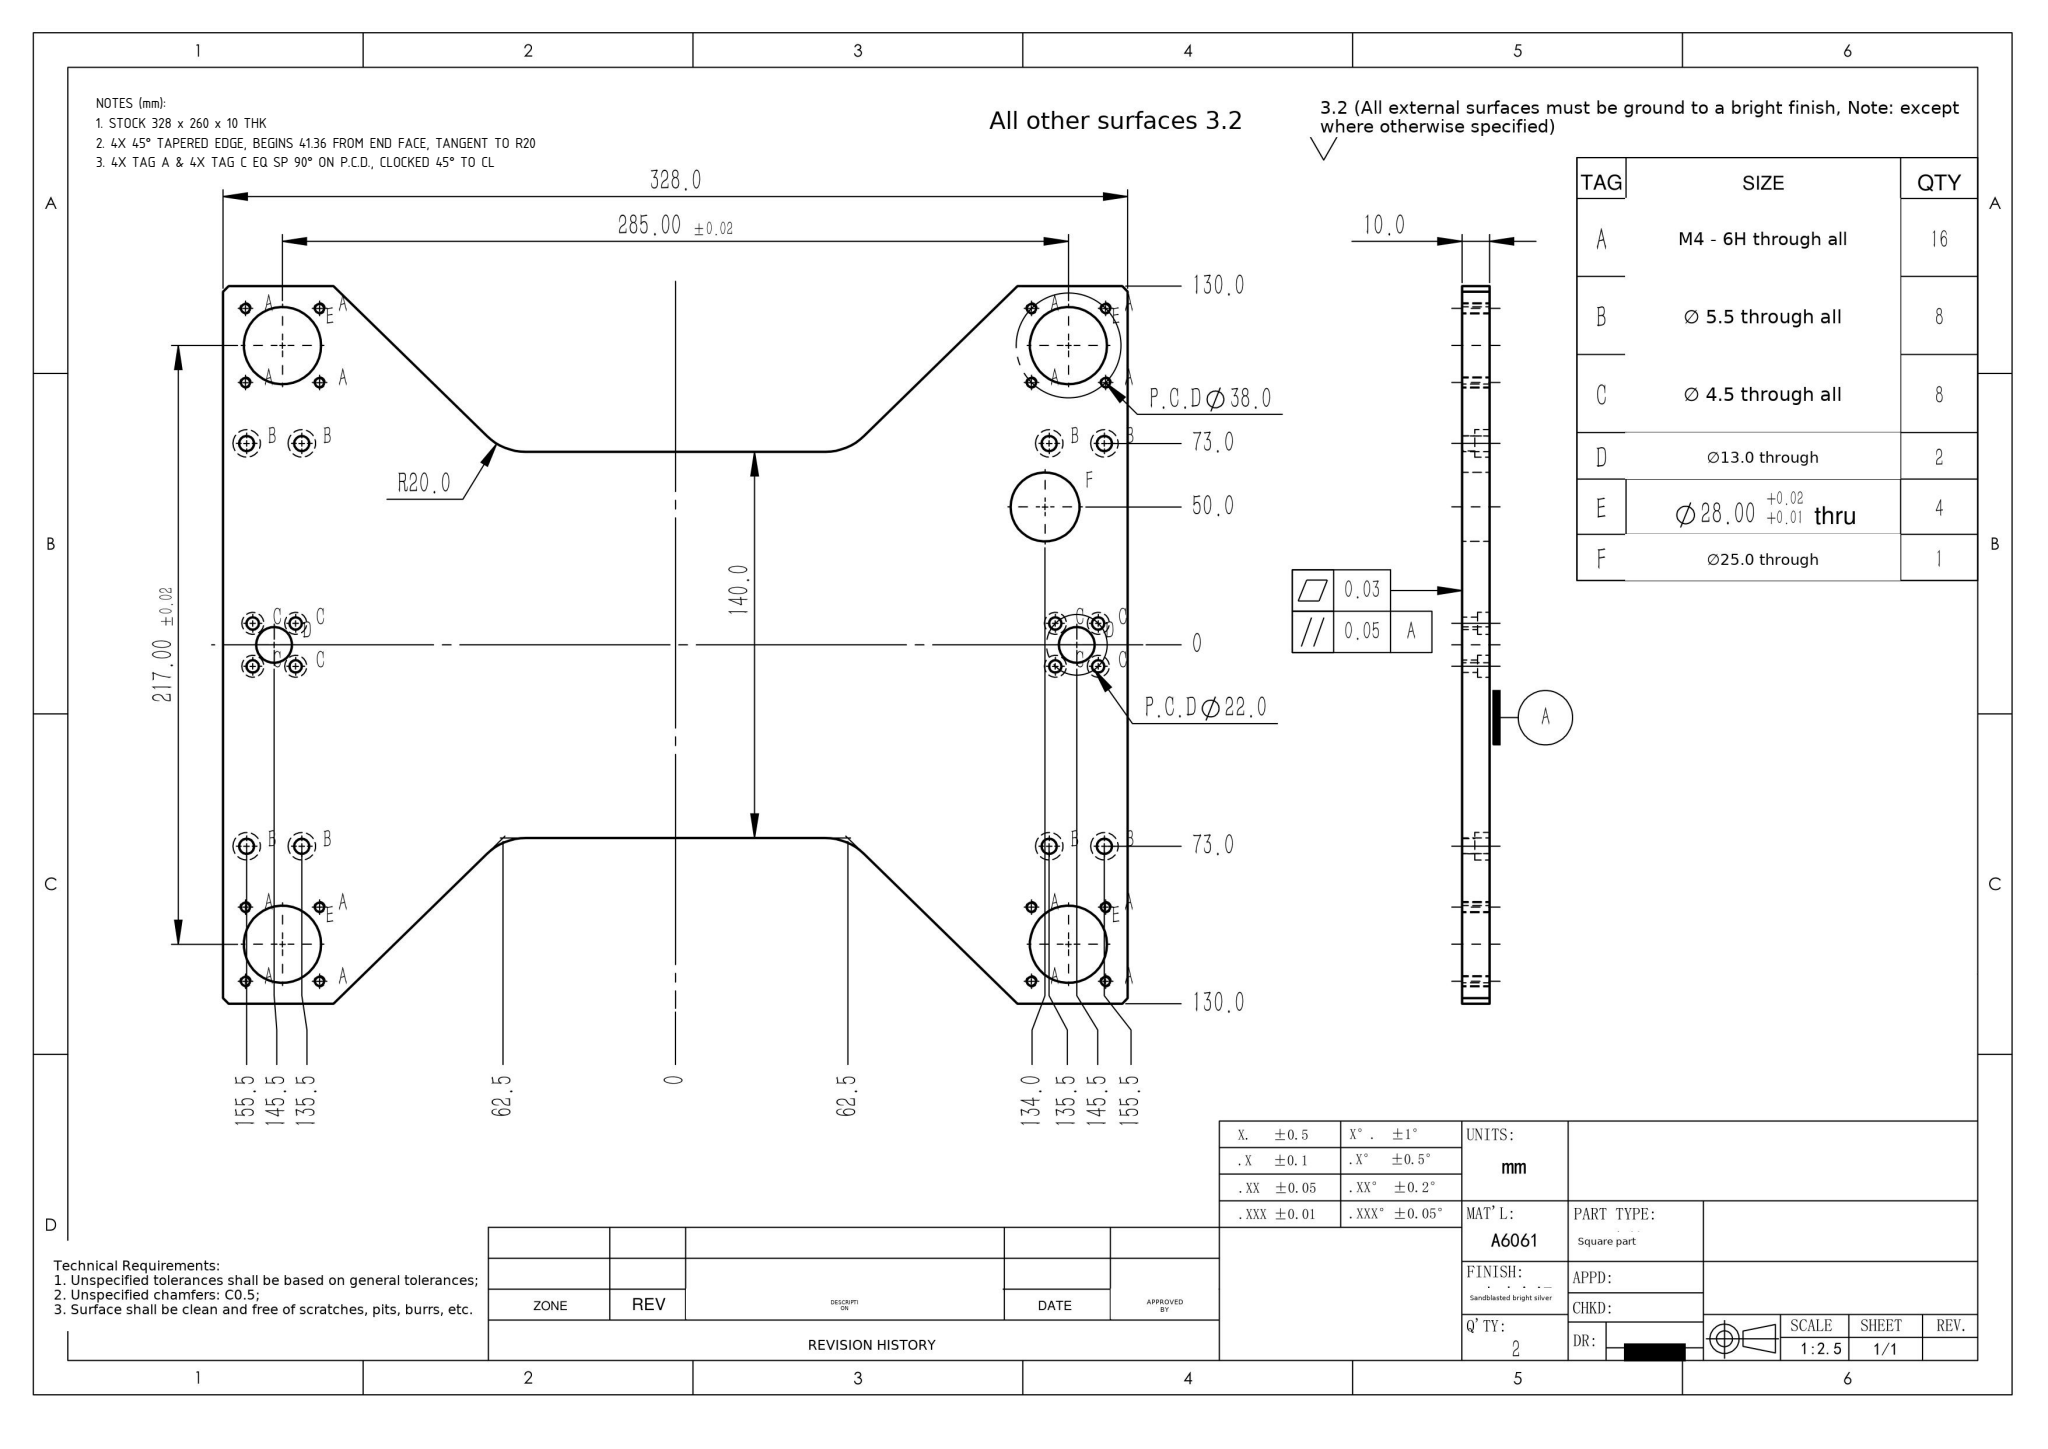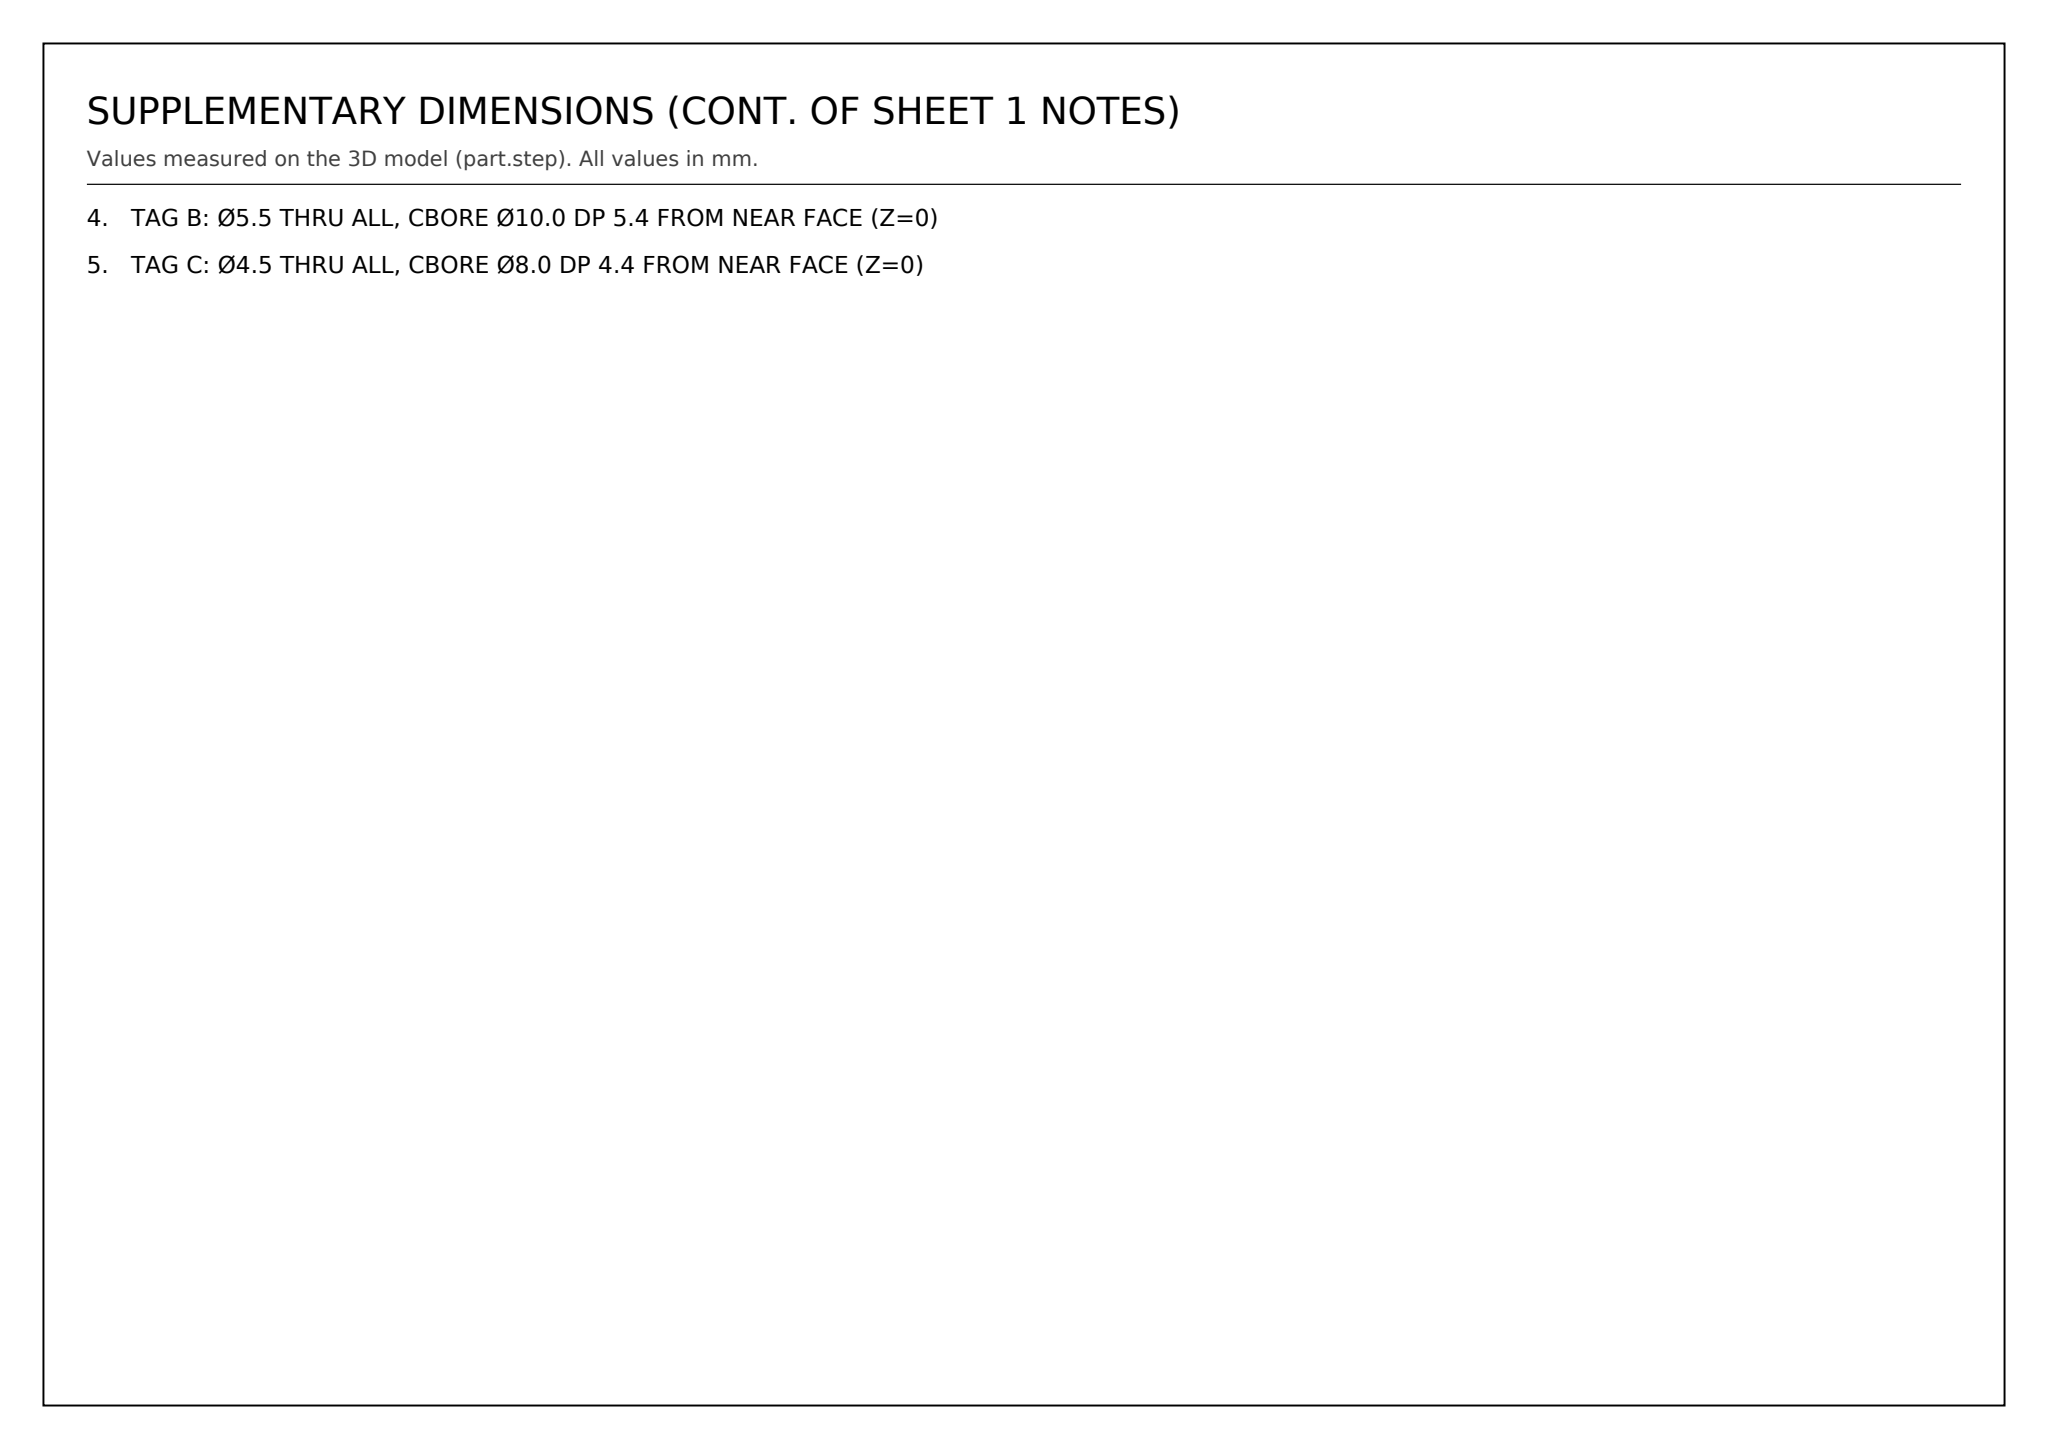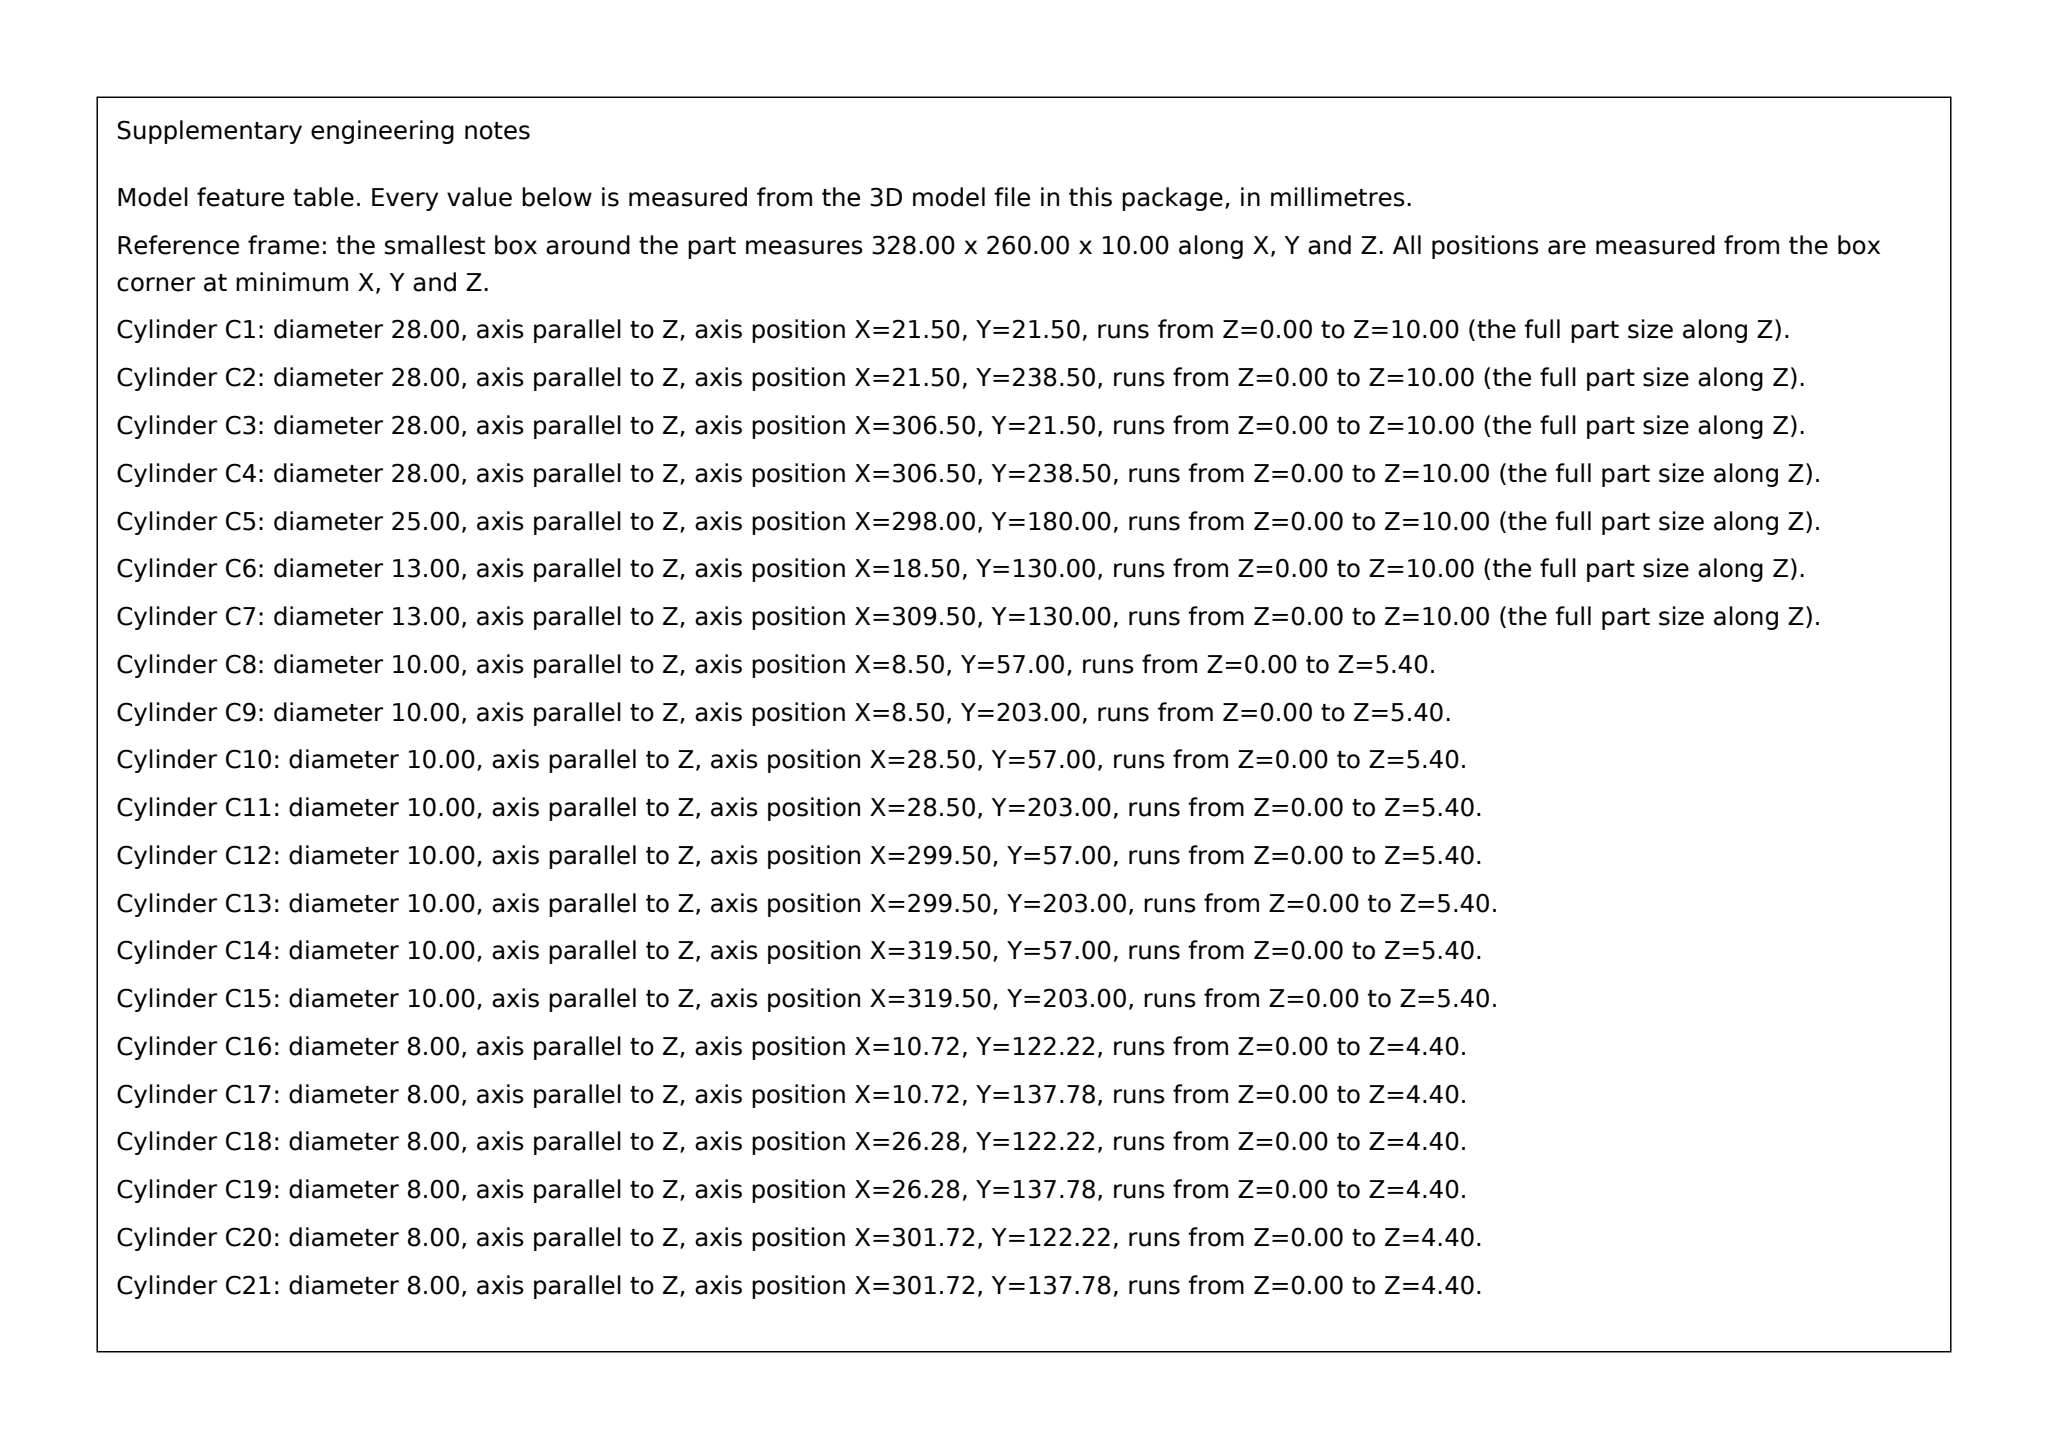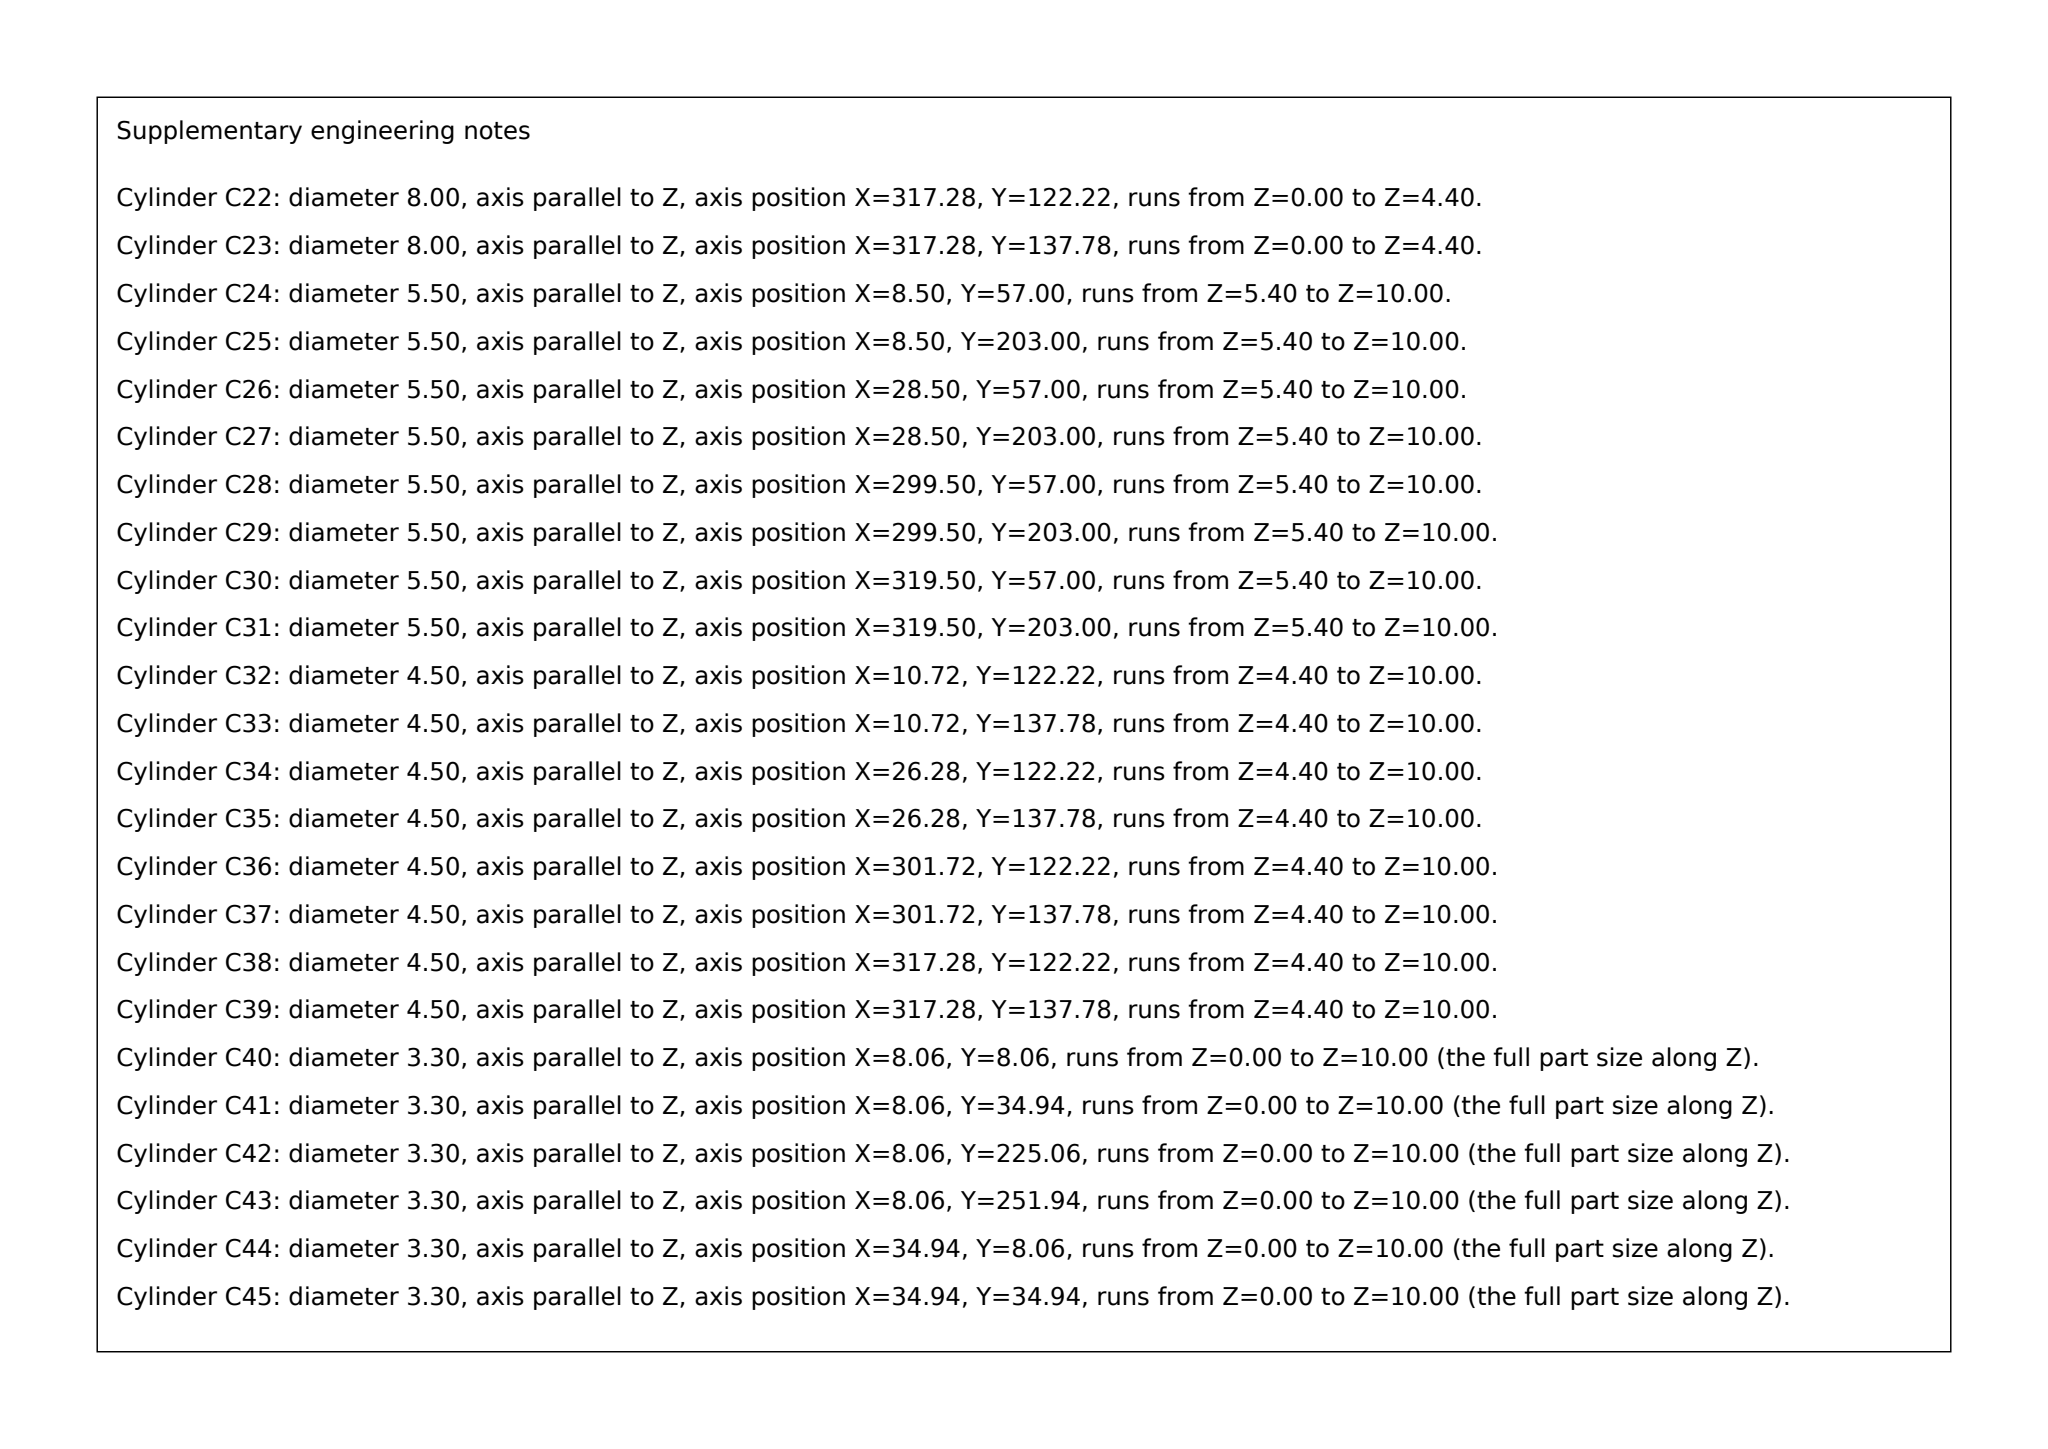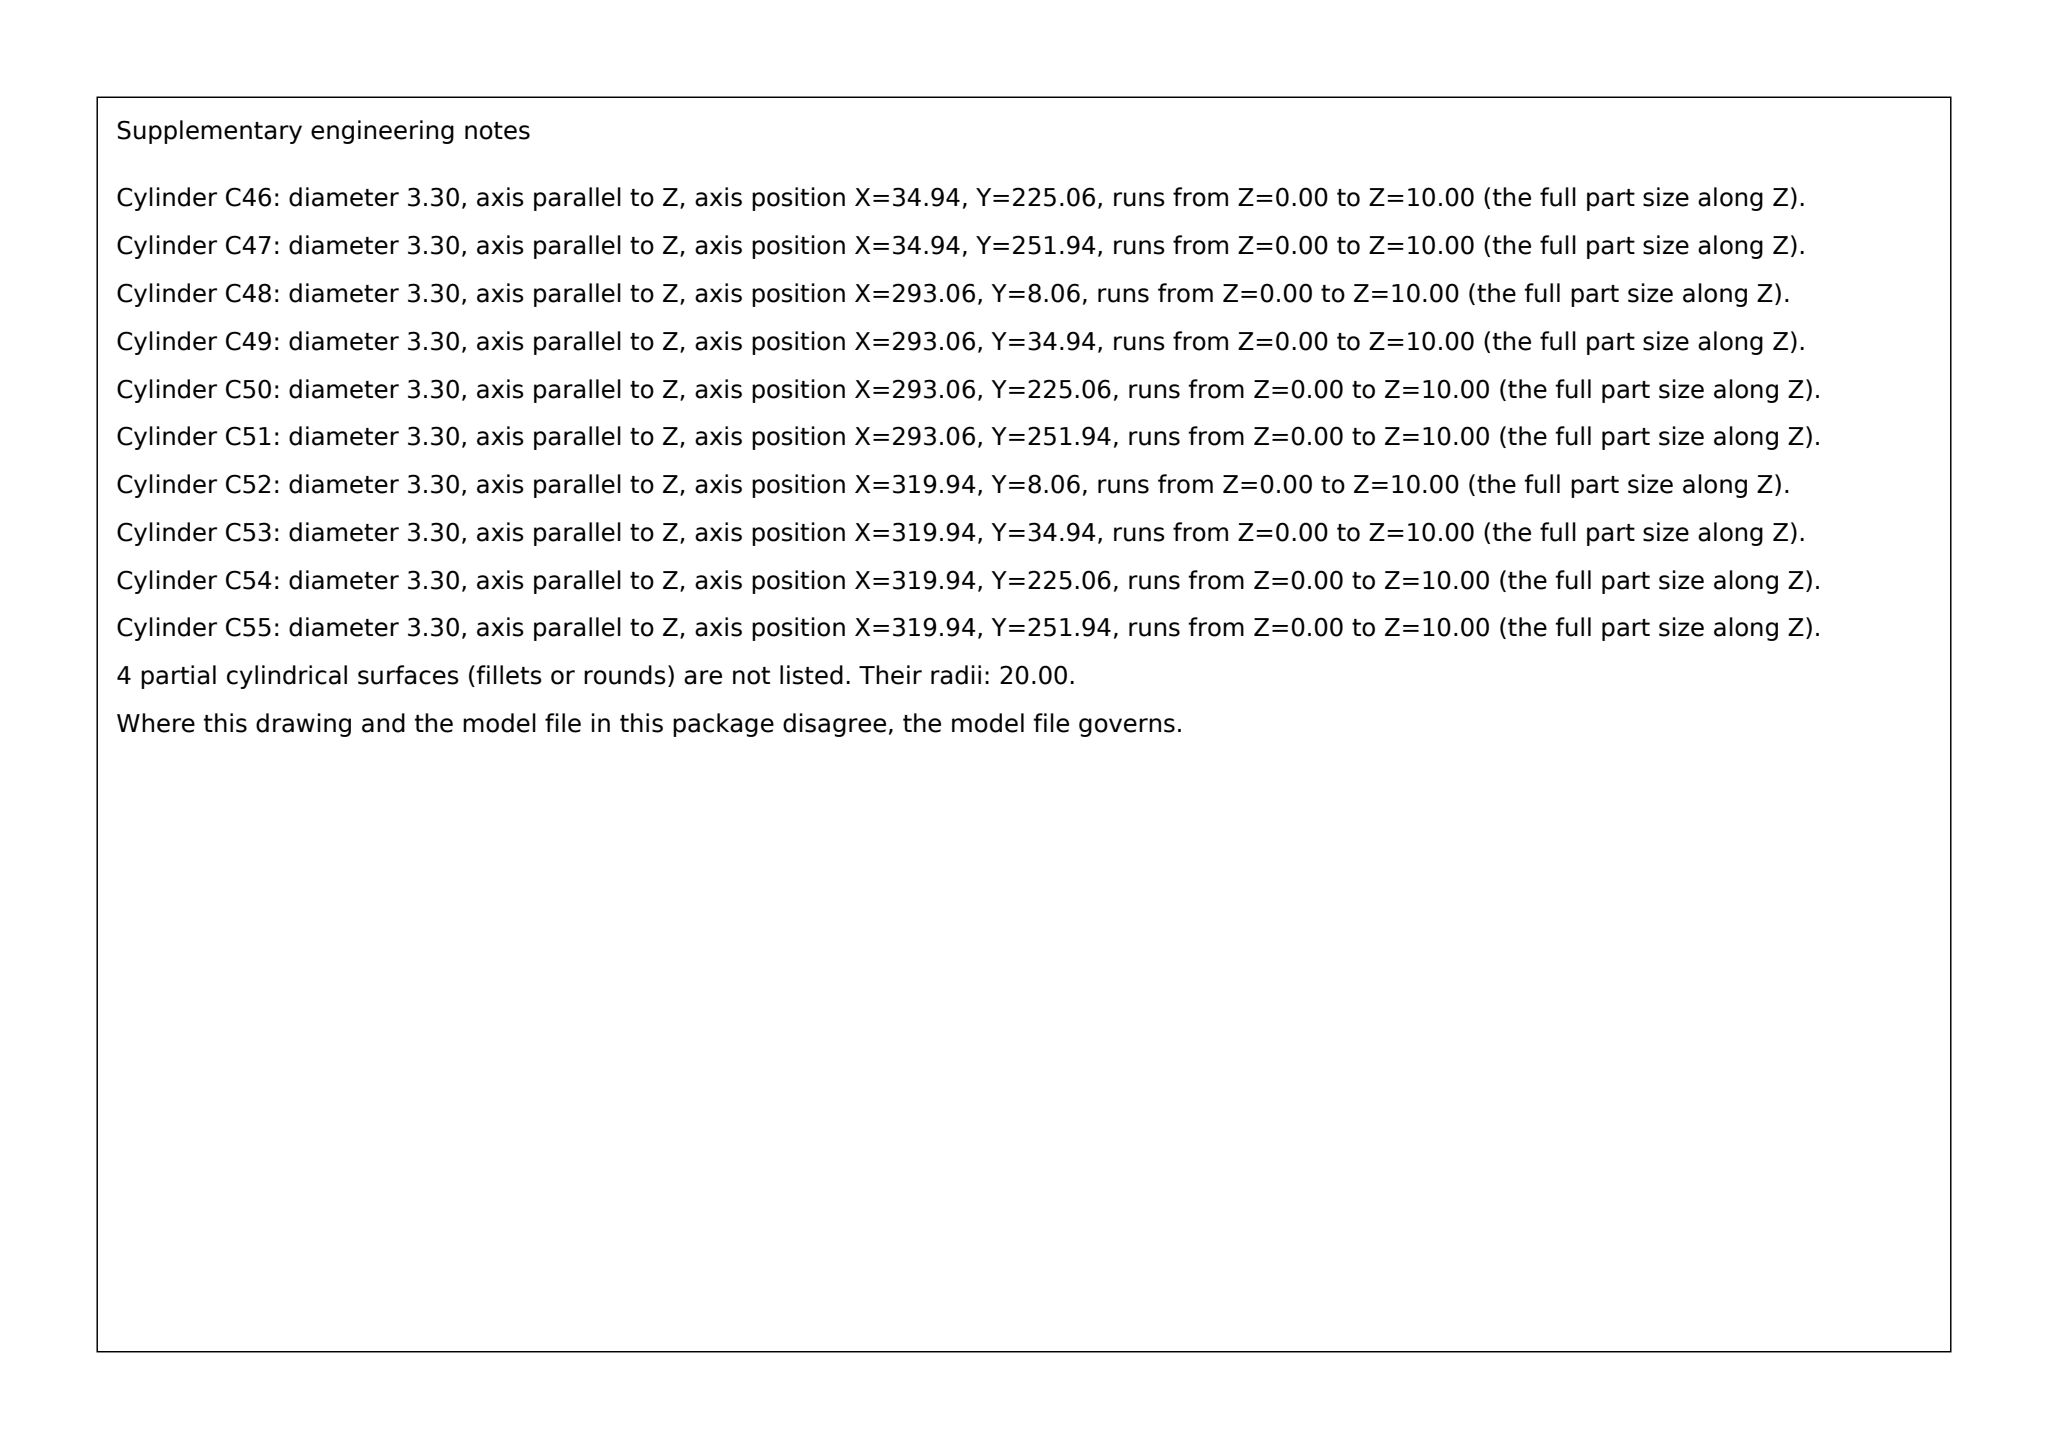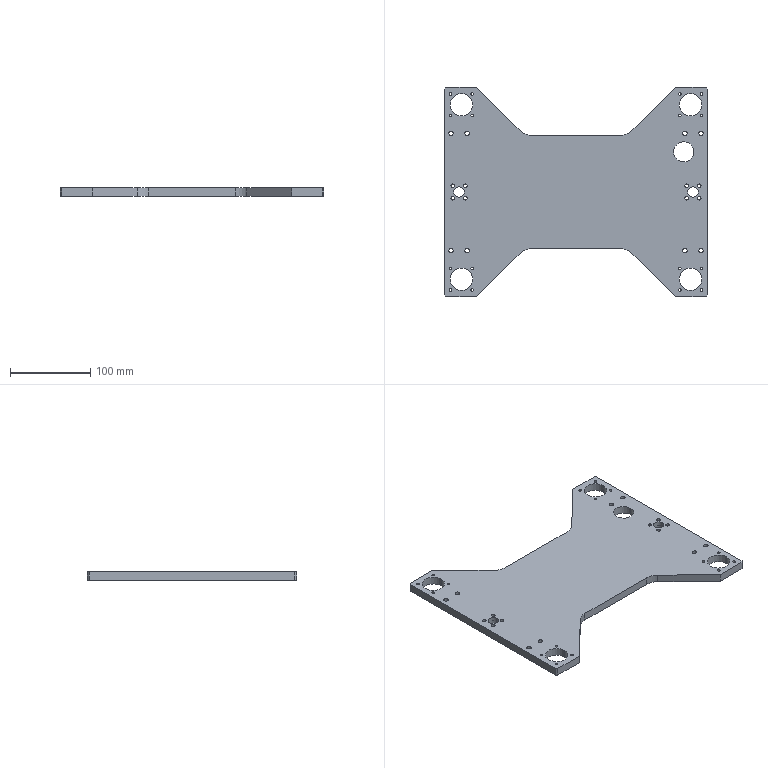Part | SolidWorks | mm | 1 solid | 148 faces | box 328 x 260 x 10 mm | volume 588937 mm3 | cylinder 114 | plane 34 | commonest cylinder face diameters 3.3 x32 8 x16 4.5 x16 10 x16 5.5 x16 28 x8 13 x4 40 x4
Drawing notes:
STOCK 328 x 260 x 10 THK | from the solid: bbox_xyz [328.0, 260.0, 10.0]; outer faces y=0 & y=260, end faces x=0 & x=328, z=0 to 10
4X 45° TAPERED EDGE, BEGINS 41.36 FROM END FACE, TANGENT TO R20 | from the solid: R20 fillets (Ø40 cyls) ctrs x=109.64/218.36, y=40/220, tangent to neck faces y=60 & y=200; 45° line meets y=0/260 at x=41.36 and 286.64
4X TAG A & 4X TAG C EQ SP 90° ON P.C.D., CLOCKED 45° TO CL | from the solid: TAG A ±13.44,±13.44 abt ctr (21.5,21.5) = R19.0 at 45°; TAG C ±7.78,±7.78 abt ctr (18.5,130) = R11.0 at 45°
TAG B: Ø5.5 THRU ALL, CBORE Ø10.0 DP 5.4 FROM NEAR FACE (Z=0) | from the solid: Ø10.0 cyl L=5.4 coaxial with Ø5.5 L=4.6 at (8.5/28.5/299.5/319.5, 57/203); z-plane 5.4 x8 = c'bore floor from z=0 face
TAG C: Ø4.5 THRU ALL, CBORE Ø8.0 DP 4.4 FROM NEAR FACE (Z=0) | from the solid: Ø8.0 cyl L=4.4 coaxial with Ø4.5 L=5.6 at (10.72/26.28/301.72/317.28, 122.22/137.78); z-plane 4.4 x8 = c'bore floor from z=0 face
build123d program:
from build123d import *

# Parameters (mm, degrees)
SKETCH1_W                                       = 328
SKETCH1_H                                       = 260
BOSS_EXTRUDE1_DEPTH                             = 10
CUT_EXTRUDE1_DEPTH                              = 210.514
SKETCH7_R                                       = 14
CUT_EXTRUDE2_DEPTH                              = 210.514
M4_TAPPED_HOLE1_D                               = 3.3
M5_HEX_SOCKET_HEAD_CAP_SCREW_CBORE1_D           = 5.5
M5_HEX_SOCKET_HEAD_CAP_SCREW_CBORE1_CBORE_D     = 10
M5_HEX_SOCKET_HEAD_CAP_SCREW_CBORE1_CBORE_DEPTH = 5.4
M4_HEX_SOCKET_HEAD_CAP_SCREW_CBORE1_D           = 4.5
M4_HEX_SOCKET_HEAD_CAP_SCREW_CBORE1_CBORE_D     = 8
M4_HEX_SOCKET_HEAD_CAP_SCREW_CBORE1_CBORE_DEPTH = 4.4
SKETCH12_R                                      = 6.5
CUT_EXTRUDE3_DEPTH                              = 210.514
SKETCH13_R                                      = 12.5
CUT_EXTRUDE4_DEPTH                              = 210.514
FILLET1_R                                       = 20
CHAMFER1_SIZE                                   = 2


with BuildPart() as part:
    # Sketch1 → Boss-Extrude1 (new body)
    with BuildSketch(Plane.XY):
        Rectangle(SKETCH1_W, SKETCH1_H)
    extrude(amount=BOSS_EXTRUDE1_DEPTH)

    # Sketch4 → Cut-Extrude1 (cut, through all)
    with BuildSketch(Plane.XY.offset(10)):
        Polygon((-124, 130), (-62.5, 70), (62.5, 70), (124, 130), align=None)
        Polygon((-124, -130), (-62.5, -70), (62.5, -70), (124, -130), align=None)
    extrude(amount=-CUT_EXTRUDE1_DEPTH, mode=Mode.SUBTRACT)

    # Sketch7 → Cut-Extrude2 (cut, through all)
    with BuildSketch(Plane.XY.offset(10)):
        with Locations((-142.5, 108.5)):
            Circle(SKETCH7_R)
        with Locations((142.5, 108.5)):
            Circle(SKETCH7_R)
        with Locations((142.5, -108.5)):
            Circle(SKETCH7_R)
        with Locations((-142.5, -108.5)):
            Circle(SKETCH7_R)
    extrude(amount=-CUT_EXTRUDE2_DEPTH, mode=Mode.SUBTRACT)

    # M4 Tapped Hole1 (through all)
    with Locations(Plane(origin=(0, 0, 0), x_dir=(-1, 0, 0), z_dir=(0, 0, -1))):
        with Locations((129.065, 95.065), (129.065, 121.935), (155.935, 121.935), (155.935, 95.065), (-129.065, 95.065), (-155.935, 95.065), (-129.065, 121.935), (-155.935, 121.935), (129.065, -95.065), (155.935, -95.065), (129.065, -121.935), (155.935, -121.935), (-155.935, -121.935), (-129.065, -121.935), (-155.935, -95.065), (-129.065, -95.065)):
            Hole(M4_TAPPED_HOLE1_D / 2)

    # M5 Hex Socket Head Cap Screw CBORE1 (through all)
    with Locations(Plane(origin=(0, 0, 0), x_dir=(-1, 0, 0), z_dir=(0, 0, -1))):
        with Locations((135.5, -73), (155.5, -73), (155.5, 73), (135.5, 73), (-135.5, 73), (-155.5, 73), (-155.5, -73), (-135.5, -73)):
            CounterBoreHole(M5_HEX_SOCKET_HEAD_CAP_SCREW_CBORE1_D / 2, M5_HEX_SOCKET_HEAD_CAP_SCREW_CBORE1_CBORE_D / 2, M5_HEX_SOCKET_HEAD_CAP_SCREW_CBORE1_CBORE_DEPTH)

    # M4 Hex Socket Head Cap Screw CBORE1 (through all)
    with Locations(Plane(origin=(0, 0, 0), x_dir=(-1, 0, 0), z_dir=(0, 0, -1))):
        with Locations((137.722, 7.778), (137.722, -7.778), (153.278, -7.778), (153.278, 7.778), (-153.278, -7.778), (-137.722, -7.778), (-153.278, 7.778), (-137.722, 7.778)):
            CounterBoreHole(M4_HEX_SOCKET_HEAD_CAP_SCREW_CBORE1_D / 2, M4_HEX_SOCKET_HEAD_CAP_SCREW_CBORE1_CBORE_D / 2, M4_HEX_SOCKET_HEAD_CAP_SCREW_CBORE1_CBORE_DEPTH)

    # Sketch12 → Cut-Extrude3 (cut, through all)
    with BuildSketch(Plane(origin=(0, 0, 0), x_dir=(-1, 0, 0), z_dir=(0, 0, -1))):
        with Locations((-145.5, 0)):
            Circle(SKETCH12_R)
        with Locations((145.5, 0)):
            Circle(SKETCH12_R)
    extrude(amount=-CUT_EXTRUDE3_DEPTH, mode=Mode.SUBTRACT)

    # Sketch13 → Cut-Extrude4 (cut, through all)
    with BuildSketch(Plane(origin=(0, 0, 0), x_dir=(-1, 0, 0), z_dir=(0, 0, -1))):
        with Locations((-134, 50)):
            Circle(SKETCH13_R)
    extrude(amount=-CUT_EXTRUDE4_DEPTH, mode=Mode.SUBTRACT)

    # Fillet1
    fillet1_edges = [part.edges().sort_by_distance(p)[0] for p in [
        (62.5, 70, 5),
        (-62.5, 70, 5),
        (-62.5, -70, 5),
        (62.5, -70, 5),
    ]]
    fillet(fillet1_edges, radius=FILLET1_R)

    # Chamfer1
    chamfer1_edges = [part.edges().sort_by_distance(p)[0] for p in [
        (164, -130, 5),
        (-164, -130, 5),
        (-164, 130, 5),
        (164, 130, 5),
    ]]
    chamfer(chamfer1_edges, length=CHAMFER1_SIZE)


solid = part.part